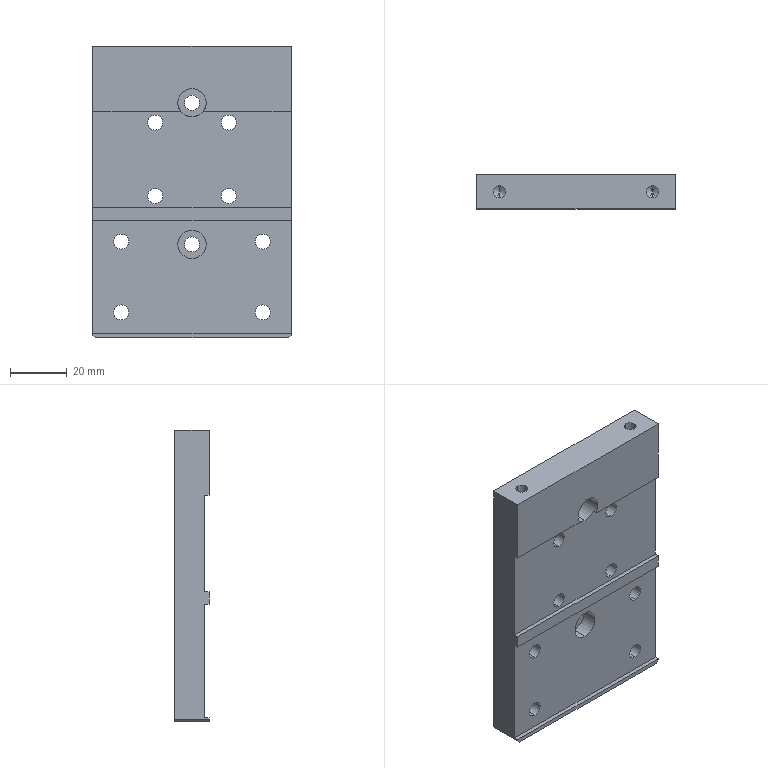Component | SolidWorks | HandlingMechanism-2_A0110-1 | 1 solid | 75 faces | box 70 x 12 x 103 mm | volume 72871 mm3 | cylinder 44 | plane 27 | cone 4 | commonest cylinder face diameters 10 x20 5.3 x20 4.2 x4
build123d program:
from build123d import *

# Parameters (mm, degrees)
SKETCH1_W                                       = 103
SKETCH1_H                                       = 70
BOSS_EXTRUDE1_DEPTH                             = 12
SKETCH6_W                                       = 40
SKETCH6_H                                       = 70
SKETCH6_W_2                                     = 34
CUT_EXTRUDE1_DEPTH                              = 1.5
M5_HEX_SOCKET_HEAD_CAP_SCREW_CBORE4_AT_2_COUNT  = 2
M5_HEX_SOCKET_HEAD_CAP_SCREW_CBORE4_AT_2_PITCH  = 50
M5_TAPPED_HOLE1_D                               = 4.2
M5_TAPPED_HOLE1_DEPTH                           = 14
M5_TAPPED_HOLE1_TIP                             = 1.262
CUT_EXTRUDE2_START                              = 10
SKETCH11_R                                      = 5
CUT_EXTRUDE2_DEPTH                              = 10
M5_HEX_SOCKET_HEAD_CAP_SCREW_CBORE6_D           = 5.3
M5_HEX_SOCKET_HEAD_CAP_SCREW_CBORE6_CBORE_D     = 10
M5_HEX_SOCKET_HEAD_CAP_SCREW_CBORE6_CBORE_DEPTH = 5.4
M5_HEX_SOCKET_HEAD_CAP_SCREW_CBORE5_D           = 5.3
M5_HEX_SOCKET_HEAD_CAP_SCREW_CBORE5_CBORE_D     = 10
M5_HEX_SOCKET_HEAD_CAP_SCREW_CBORE5_CBORE_DEPTH = 5.4
CHAMFER1_SIZE                                   = 1


with BuildPart() as part:
    # Sketch1 → Boss-Extrude1 (new body)
    with BuildSketch(Plane.XY):
        Rectangle(SKETCH1_W, SKETCH1_H)
    extrude(amount=BOSS_EXTRUDE1_DEPTH)

    # Sketch6 → Cut-Extrude1 (cut)
    with BuildSketch(Plane(origin=(0, 0, 0), x_dir=(-1, 0, 0), z_dir=(0, 0, -1))):
        with Locations((30, 0)):
            Rectangle(SKETCH6_W, SKETCH6_H)
        with Locations((-11.5, 0)):
            Rectangle(SKETCH6_W_2, SKETCH6_H)
    extrude(amount=-CUT_EXTRUDE1_DEPTH, mode=Mode.SUBTRACT)

    # Sketch7 → M5 Hex Socket Head Cap Screw CBORE4 (revolve, cut)
    with BuildSketch(Plane(origin=(31.5, 0, 1.5), x_dir=(0, 1, 0), z_dir=(1, 0, 0))):
        Polygon((0, 0), (0, 10.5), (2.65, 10.5), (2.65, 5.4), (5, 5.4), (5, 0), align=None)
    m5_hex_socket_head_cap_screw_cbore4 = revolve(axis=Axis((31.5, 0, -4.85), (0, 0, 1)), mode=Mode.SUBTRACT)

    # M5 Hex Socket Head Cap Screw CBORE4 at 2: M5 Hex Socket Head Cap Screw CBORE4 ×2
    with Locations(*[(-i * M5_HEX_SOCKET_HEAD_CAP_SCREW_CBORE4_AT_2_PITCH, 0, 0) for i in range(1, M5_HEX_SOCKET_HEAD_CAP_SCREW_CBORE4_AT_2_COUNT)]):
        add(m5_hex_socket_head_cap_screw_cbore4, mode=Mode.SUBTRACT)

    # M5 Tapped Hole1
    with Locations(Plane(origin=(51.5, 0, 0), x_dir=(0, 0, -1), z_dir=(1, 0, 0))):
        with Locations((-6, 27), (-6, -27)):
            Hole(M5_TAPPED_HOLE1_D / 2, depth=M5_TAPPED_HOLE1_DEPTH)
            with Locations((0, 0, -(M5_TAPPED_HOLE1_DEPTH + M5_TAPPED_HOLE1_TIP / 2))):  # 118° drill point
                Cone(0, M5_TAPPED_HOLE1_D / 2, M5_TAPPED_HOLE1_TIP, mode=Mode.SUBTRACT)

    # Sketch11 → Cut-Extrude2 (cut)
    with BuildSketch(Plane(origin=(0, 0, 6.9), x_dir=(-1, 0, 0), z_dir=(0, 0, -1)).offset(CUT_EXTRUDE2_START)):
        with Locations((-31.5, 0)):
            Circle(SKETCH11_R)
    extrude(amount=-CUT_EXTRUDE2_DEPTH, mode=Mode.SUBTRACT)

    # M5 Hex Socket Head Cap Screw CBORE6 (through all)
    with Locations(Plane.XY.offset(12)):
        with Locations((-1.5, -13), (24.5, -13), (24.5, 13), (-1.5, 13)):
            CounterBoreHole(M5_HEX_SOCKET_HEAD_CAP_SCREW_CBORE6_D / 2, M5_HEX_SOCKET_HEAD_CAP_SCREW_CBORE6_CBORE_D / 2, M5_HEX_SOCKET_HEAD_CAP_SCREW_CBORE6_CBORE_DEPTH)

    # M5 Hex Socket Head Cap Screw CBORE5 (through all)
    with Locations(Plane.XY.offset(12)):
        with Locations((-42.5, 25), (-17.5, 25), (-17.5, -25), (-42.5, -25)):
            CounterBoreHole(M5_HEX_SOCKET_HEAD_CAP_SCREW_CBORE5_D / 2, M5_HEX_SOCKET_HEAD_CAP_SCREW_CBORE5_CBORE_D / 2, M5_HEX_SOCKET_HEAD_CAP_SCREW_CBORE5_CBORE_DEPTH)

    # Chamfer1
    chamfer1_edges = [part.edges().sort_by_distance(p)[0] for p in [
        (-51.5, -35, 6),
        (-51.5, 35, 6),
    ]]
    chamfer(chamfer1_edges, length=CHAMFER1_SIZE)


solid = part.part

# Placed as in the assembly
solid = solid.moved(Location((25.881, 39.5, 71.5), (-90, 0, -90)))